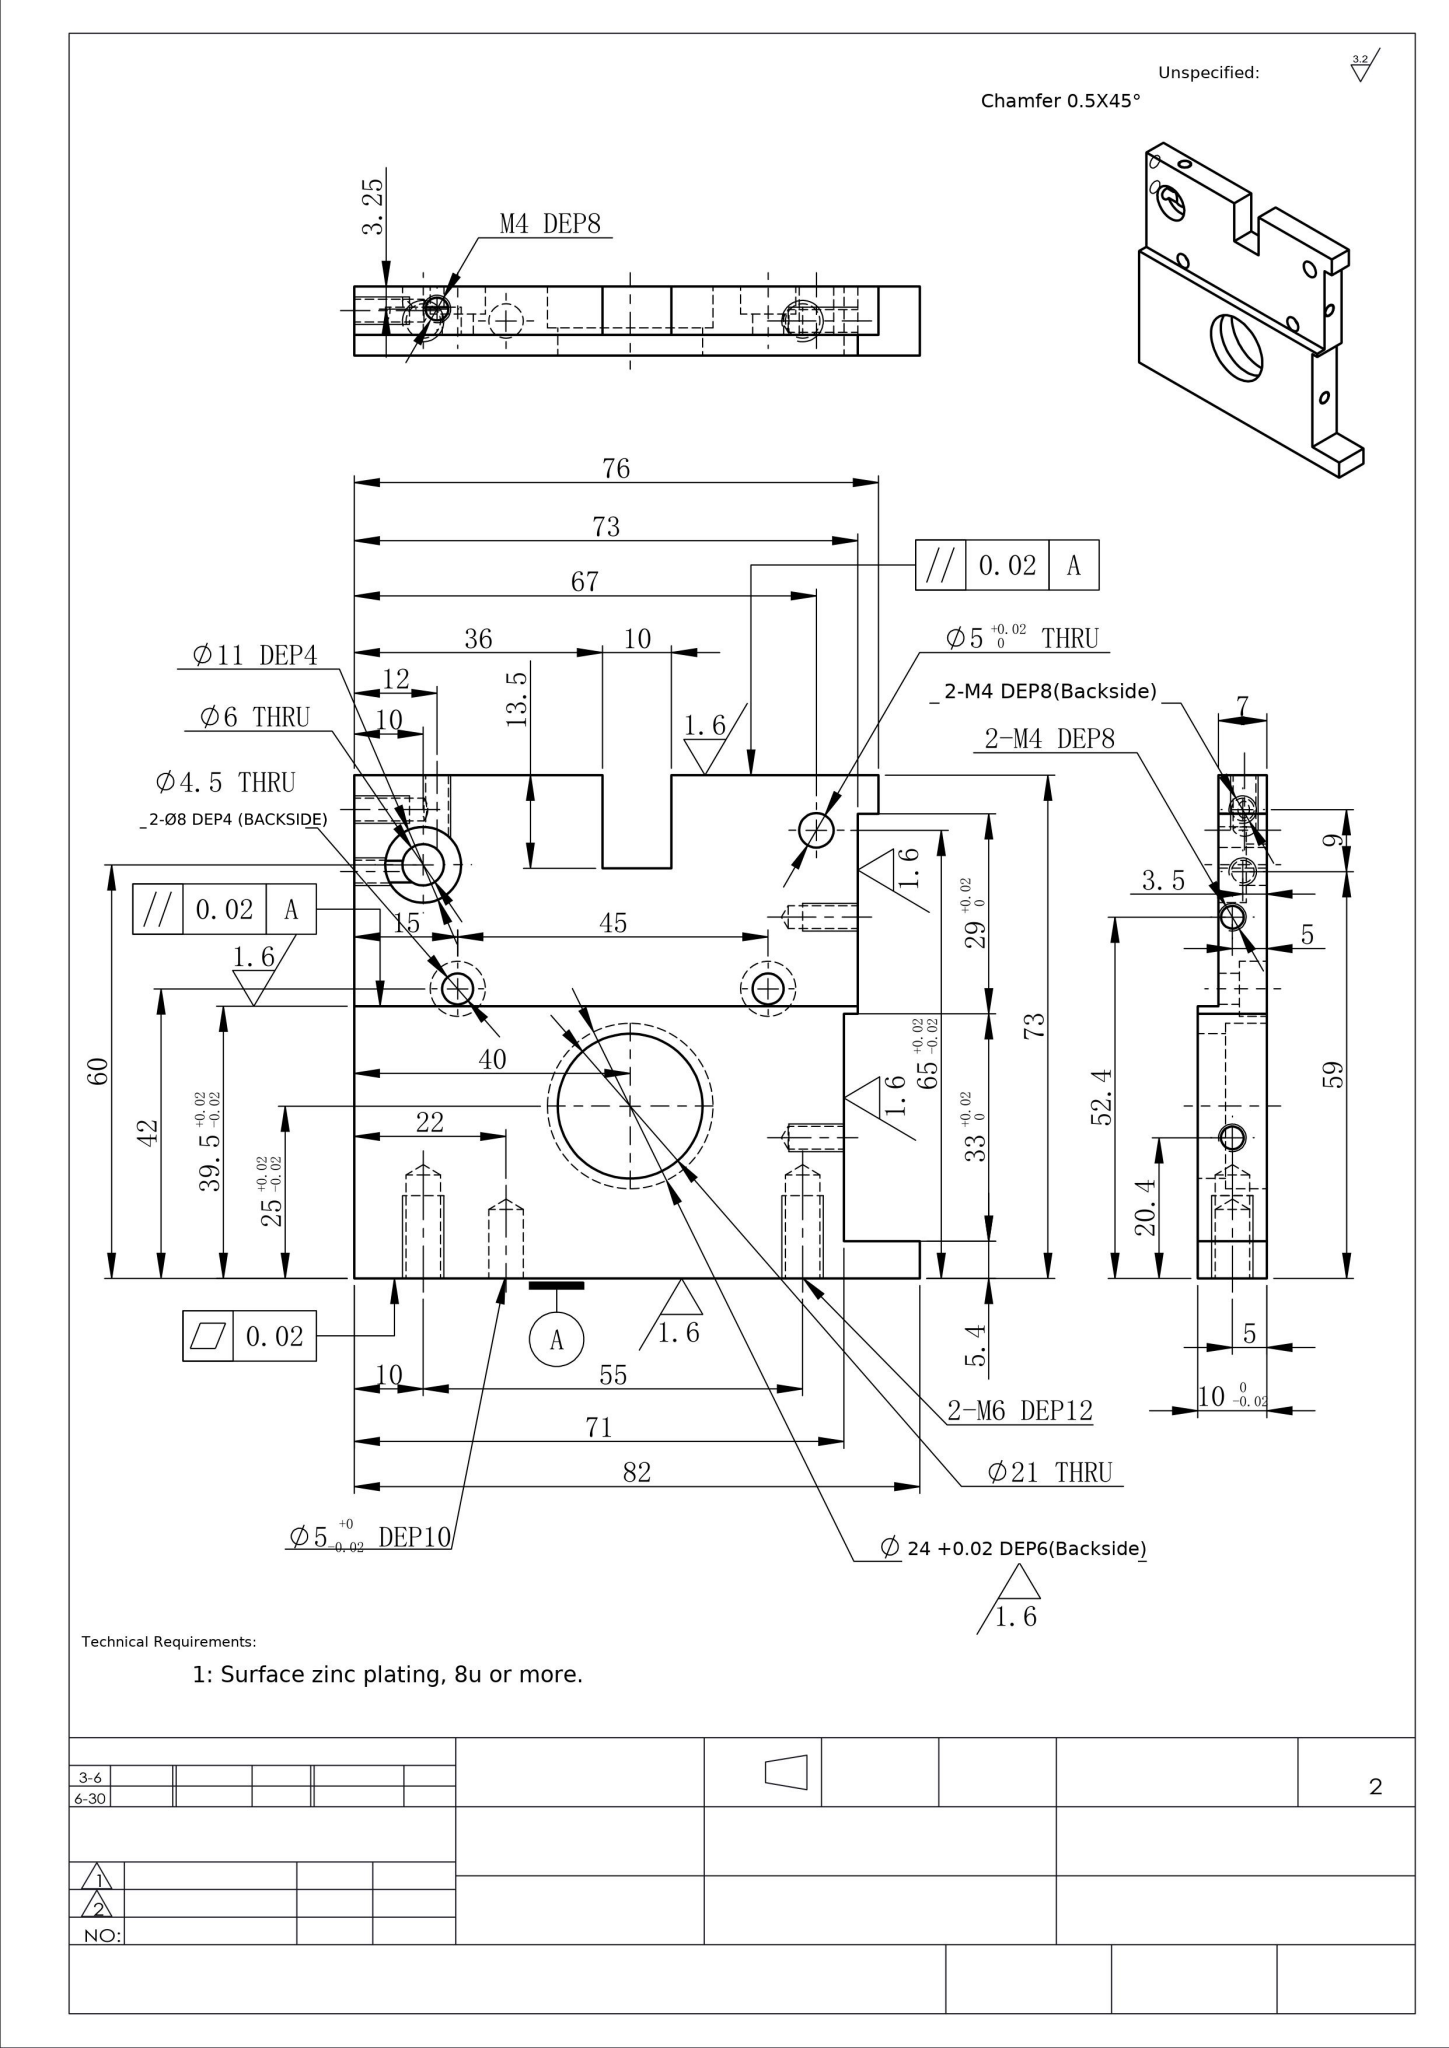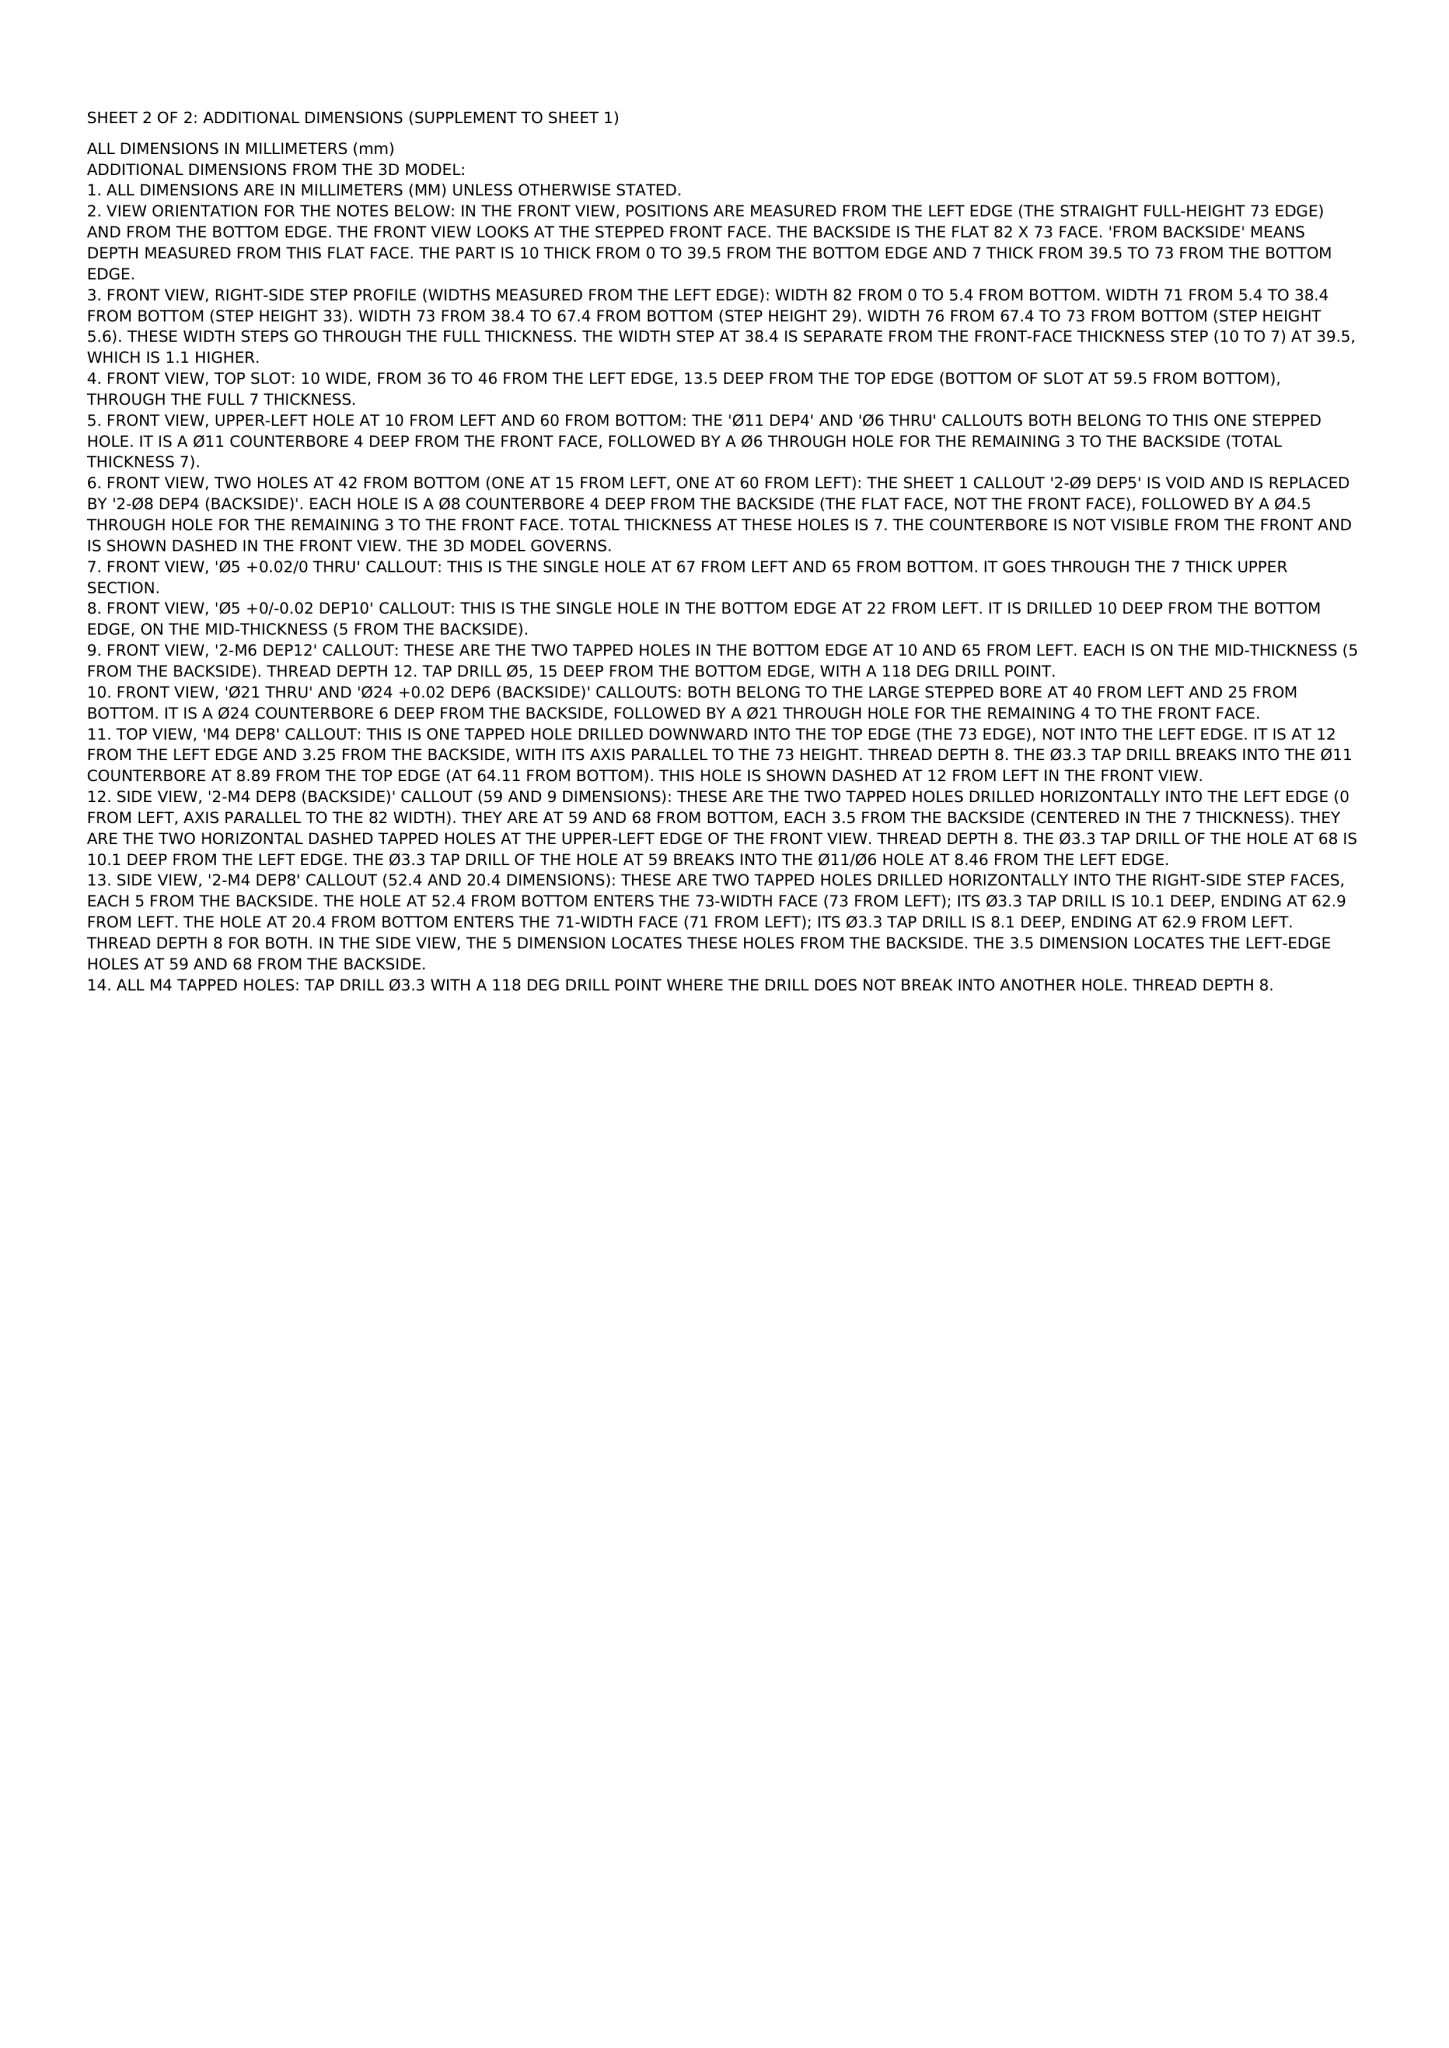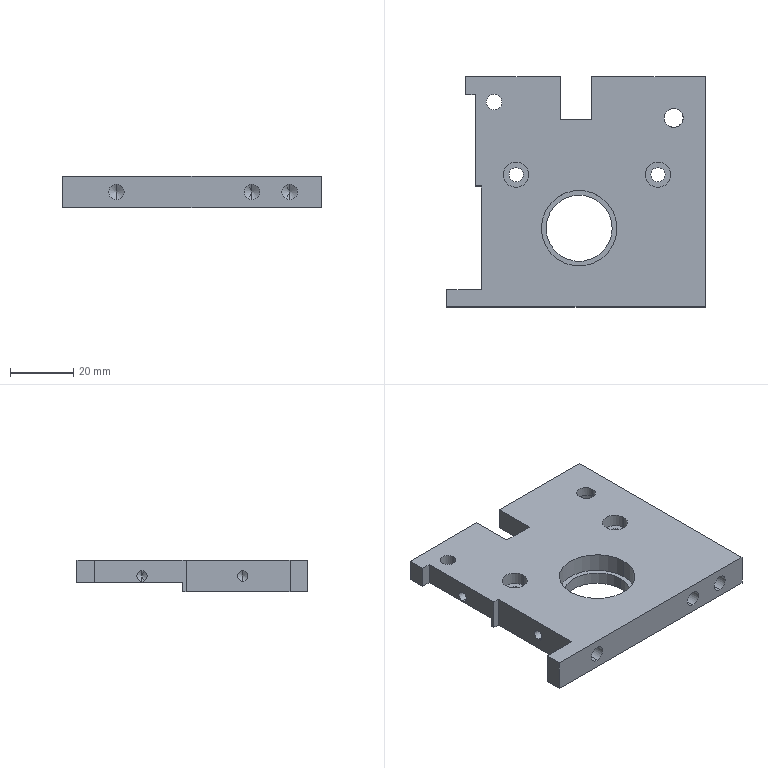Part | NX | mm | Counterbored Square Mounting Plate 73mm | 1 solid | 69 faces | box 82 x 73 x 10 mm | volume 38573 mm3 | cylinder 35 | plane 22 | cone 12 | commonest cylinder face diameters 3.3 x10 5 x8 4.5 x4 8 x4 11 x3 21 x2 24 x2 6 x2